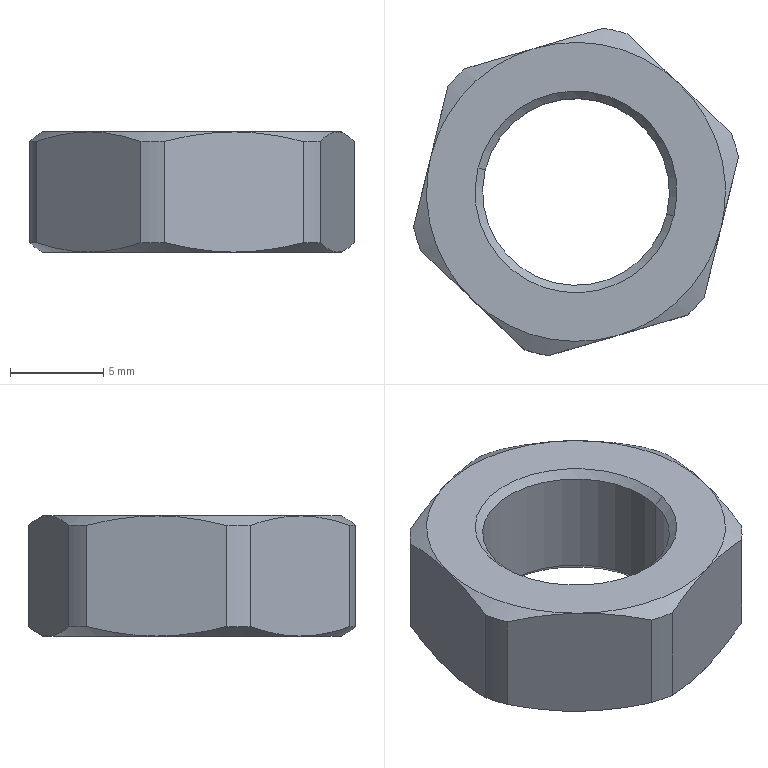Component | SolidWorks | ControlAssembly-1_UWAFN120-1_3_1-1 | 1 solid | 32 faces | box 17.38 x 17.53 x 6.43 mm | volume 899 mm3 | cone 16 | cylinder 8 | plane 8 | commonest cylinder face diameters 17.77 x6 10.002 x2
STEP:
#1=CARTESIAN_POINT('',(24.816,0.7631,20.553));
#2=VERTEX_POINT('',#1);
#3=CARTESIAN_POINT('',(24.433,0.8563,20.553));
#4=VERTEX_POINT('',#3);
#5=CARTESIAN_POINT('',(24.624,0.8097,20.553));
#6=DIRECTION('',(-0.00009864,0.,-1.));
#7=DIRECTION('',(-0.9716,0.2366,0.00009584));
#8=AXIS2_PLACEMENT_3D('',#5,#6,#7);
#9=CIRCLE('',#8,0.1969);
#10=EDGE_CURVE('',#2,#4,#9,.T.);
#11=ORIENTED_EDGE('',*,*,#10,.T.);
#12=CARTESIAN_POINT('',(24.418,0.86,20.569));
#13=VERTEX_POINT('',#12);
#14=CARTESIAN_POINT('',(24.433,0.8563,20.553));
#15=DIRECTION('',(-0.687,0.1673,0.7072));
#16=VECTOR('',#15,39.37);
#17=LINE('',#14,#16);
#18=EDGE_CURVE('',#4,#13,#17,.T.);
#19=ORIENTED_EDGE('',*,*,#18,.T.);
#20=CARTESIAN_POINT('',(24.831,0.7594,20.569));
#21=VERTEX_POINT('',#20);
#22=CARTESIAN_POINT('',(24.624,0.8097,20.569));
#23=DIRECTION('',(0.00009864,-0.,1.));
#24=DIRECTION('',(0.9716,-0.2366,-0.00009584));
#25=AXIS2_PLACEMENT_3D('',#22,#23,#24);
#26=CIRCLE('',#25,0.2126);
#27=EDGE_CURVE('',#13,#21,#26,.T.);
#28=ORIENTED_EDGE('',*,*,#27,.T.);
#29=CARTESIAN_POINT('',(24.816,0.7631,20.553));
#30=DIRECTION('',(0.6871,-0.1673,0.707));
#31=VECTOR('',#30,39.37);
#32=LINE('',#29,#31);
#33=EDGE_CURVE('',#2,#21,#32,.T.);
#34=ORIENTED_EDGE('',*,*,#33,.F.);
#35=EDGE_LOOP('',(#11,#19,#28,#34));
#36=FACE_OUTER_BOUND('',#35,.T.);
#37=CARTESIAN_POINT('',(24.624,0.8097,20.553));
#38=DIRECTION('',(0.00009864,-0.,1.));
#39=DIRECTION('',(0.9716,-0.2366,-0.00009584));
#40=AXIS2_PLACEMENT_3D('',#37,#38,#39);
#41=CONICAL_SURFACE('',#40,0.1969,0.7854);
#42=ADVANCED_FACE('',(#36),#41,.F.);
#43=ORIENTED_EDGE('',*,*,#10,.F.);
#44=CARTESIAN_POINT('',(24.816,0.7631,20.331));
#45=VERTEX_POINT('',#44);
#46=CARTESIAN_POINT('',(24.816,0.7631,20.198));
#47=DIRECTION('',(-0.00009864,0.,-1.));
#48=VECTOR('',#47,39.37);
#49=LINE('',#46,#48);
#50=EDGE_CURVE('',#2,#45,#49,.T.);
#51=ORIENTED_EDGE('',*,*,#50,.T.);
#52=CARTESIAN_POINT('',(24.433,0.8563,20.331));
#53=VERTEX_POINT('',#52);
#54=CARTESIAN_POINT('',(24.624,0.8097,20.331));
#55=DIRECTION('',(-0.00009864,0.,-1.));
#56=DIRECTION('',(-0.9716,0.2366,0.00009584));
#57=AXIS2_PLACEMENT_3D('',#54,#55,#56);
#58=CIRCLE('',#57,0.1969);
#59=EDGE_CURVE('',#45,#53,#58,.T.);
#60=ORIENTED_EDGE('',*,*,#59,.T.);
#61=CARTESIAN_POINT('',(24.433,0.8563,20.198));
#62=DIRECTION('',(-0.00009864,0.,-1.));
#63=VECTOR('',#62,39.37);
#64=LINE('',#61,#63);
#65=EDGE_CURVE('',#4,#53,#64,.T.);
#66=ORIENTED_EDGE('',*,*,#65,.F.);
#67=EDGE_LOOP('',(#43,#51,#60,#66));
#68=FACE_OUTER_BOUND('',#67,.T.);
#69=CARTESIAN_POINT('',(24.624,0.8097,20.198));
#70=DIRECTION('',(-0.00009864,0.,-1.));
#71=DIRECTION('',(-0.9716,0.2366,0.00009584));
#72=AXIS2_PLACEMENT_3D('',#69,#70,#71);
#73=CYLINDRICAL_SURFACE('',#72,0.1969);
#74=ADVANCED_FACE('',(#68),#73,.F.);
#75=ORIENTED_EDGE('',*,*,#59,.F.);
#76=CARTESIAN_POINT('',(24.831,0.7594,20.316));
#77=VERTEX_POINT('',#76);
#78=CARTESIAN_POINT('',(24.869,0.7501,20.276));
#79=DIRECTION('',(0.687,-0.1673,-0.7072));
#80=VECTOR('',#79,39.37);
#81=LINE('',#78,#80);
#82=EDGE_CURVE('',#45,#77,#81,.T.);
#83=ORIENTED_EDGE('',*,*,#82,.T.);
#84=CARTESIAN_POINT('',(24.418,0.86,20.316));
#85=VERTEX_POINT('',#84);
#86=CARTESIAN_POINT('',(24.624,0.8097,20.316));
#87=DIRECTION('',(-0.00009864,0.,-1.));
#88=DIRECTION('',(-0.9716,0.2366,0.00009584));
#89=AXIS2_PLACEMENT_3D('',#86,#87,#88);
#90=CIRCLE('',#89,0.2126);
#91=EDGE_CURVE('',#77,#85,#90,.T.);
#92=ORIENTED_EDGE('',*,*,#91,.T.);
#93=CARTESIAN_POINT('',(24.379,0.8693,20.276));
#94=DIRECTION('',(-0.6871,0.1673,-0.707));
#95=VECTOR('',#94,39.37);
#96=LINE('',#93,#95);
#97=EDGE_CURVE('',#53,#85,#96,.T.);
#98=ORIENTED_EDGE('',*,*,#97,.F.);
#99=EDGE_LOOP('',(#75,#83,#92,#98));
#100=FACE_OUTER_BOUND('',#99,.T.);
#101=CARTESIAN_POINT('',(24.624,0.8097,20.276));
#102=DIRECTION('',(-0.00009864,0.,-1.));
#103=DIRECTION('',(-0.9716,0.2366,0.00009584));
#104=AXIS2_PLACEMENT_3D('',#101,#102,#103);
#105=CONICAL_SURFACE('',#104,0.252,0.7854);
#106=ADVANCED_FACE('',(#100),#105,.F.);
#107=CARTESIAN_POINT('',(24.624,0.8097,20.316));
#108=DIRECTION('',(-0.00009864,0.,-1.));
#109=DIRECTION('',(-0.9716,0.2366,0.00009584));
#110=AXIS2_PLACEMENT_3D('',#107,#108,#109);
#111=CIRCLE('',#110,0.2126);
#112=EDGE_CURVE('',#85,#77,#111,.T.);
#113=ORIENTED_EDGE('',*,*,#112,.F.);
#114=ORIENTED_EDGE('',*,*,#91,.F.);
#115=EDGE_LOOP('',(#113,#114));
#116=FACE_BOUND('',#115,.T.);
#117=CARTESIAN_POINT('',(24.842,1.037,20.316));
#118=VERTEX_POINT('',#117);
#119=CARTESIAN_POINT('',(24.93,0.7352,20.316));
#120=VERTEX_POINT('',#119);
#121=CARTESIAN_POINT('',(24.624,0.8097,20.316));
#122=DIRECTION('',(-0.00009864,0.,-1.));
#123=DIRECTION('',(0.9716,-0.2366,-0.00009584));
#124=AXIS2_PLACEMENT_3D('',#121,#122,#123);
#125=CIRCLE('',#124,0.315);
#126=EDGE_CURVE('',#118,#120,#125,.T.);
#127=ORIENTED_EDGE('',*,*,#126,.T.);
#128=CARTESIAN_POINT('',(24.713,0.5074,20.316));
#129=VERTEX_POINT('',#128);
#130=CARTESIAN_POINT('',(24.624,0.8097,20.316));
#131=DIRECTION('',(-0.00009864,0.,-1.));
#132=DIRECTION('',(0.9716,-0.2366,-0.00009584));
#133=AXIS2_PLACEMENT_3D('',#130,#131,#132);
#134=CIRCLE('',#133,0.315);
#135=EDGE_CURVE('',#120,#129,#134,.T.);
#136=ORIENTED_EDGE('',*,*,#135,.T.);
#137=CARTESIAN_POINT('',(24.407,0.5819,20.316));
#138=VERTEX_POINT('',#137);
#139=CARTESIAN_POINT('',(24.624,0.8097,20.316));
#140=DIRECTION('',(-0.00009864,0.,-1.));
#141=DIRECTION('',(0.9716,-0.2366,-0.00009584));
#142=AXIS2_PLACEMENT_3D('',#139,#140,#141);
#143=CIRCLE('',#142,0.315);
#144=EDGE_CURVE('',#129,#138,#143,.T.);
#145=ORIENTED_EDGE('',*,*,#144,.T.);
#146=CARTESIAN_POINT('',(24.318,0.8842,20.316));
#147=VERTEX_POINT('',#146);
#148=CARTESIAN_POINT('',(24.624,0.8097,20.316));
#149=DIRECTION('',(-0.00009864,0.,-1.));
#150=DIRECTION('',(0.9716,-0.2366,-0.00009584));
#151=AXIS2_PLACEMENT_3D('',#148,#149,#150);
#152=CIRCLE('',#151,0.315);
#153=EDGE_CURVE('',#138,#147,#152,.T.);
#154=ORIENTED_EDGE('',*,*,#153,.T.);
#155=CARTESIAN_POINT('',(24.536,1.112,20.316));
#156=VERTEX_POINT('',#155);
#157=CARTESIAN_POINT('',(24.624,0.8097,20.316));
#158=DIRECTION('',(-0.00009864,0.,-1.));
#159=DIRECTION('',(0.9716,-0.2366,-0.00009584));
#160=AXIS2_PLACEMENT_3D('',#157,#158,#159);
#161=CIRCLE('',#160,0.315);
#162=EDGE_CURVE('',#147,#156,#161,.T.);
#163=ORIENTED_EDGE('',*,*,#162,.T.);
#164=CARTESIAN_POINT('',(24.624,0.8097,20.316));
#165=DIRECTION('',(-0.00009864,0.,-1.));
#166=DIRECTION('',(0.9716,-0.2366,-0.00009584));
#167=AXIS2_PLACEMENT_3D('',#164,#165,#166);
#168=CIRCLE('',#167,0.315);
#169=EDGE_CURVE('',#156,#118,#168,.T.);
#170=ORIENTED_EDGE('',*,*,#169,.T.);
#171=EDGE_LOOP('',(#127,#136,#145,#154,#163,#170));
#172=FACE_OUTER_BOUND('',#171,.T.);
#173=CARTESIAN_POINT('',(24.587,0.6567,20.316));
#174=DIRECTION('',(-0.00009864,0.,-1.));
#175=DIRECTION('',(-0.9716,0.2366,0.00009584));
#176=AXIS2_PLACEMENT_3D('',#173,#174,#175);
#177=PLANE('',#176);
#178=ADVANCED_FACE('',(#116,#172),#177,.T.);
#179=CARTESIAN_POINT('',(24.859,0.5502,20.336));
#180=VERTEX_POINT('',#179);
#181=CARTESIAN_POINT('',(24.859,0.5502,20.336));
#182=CARTESIAN_POINT('',(24.811,0.5361,20.323));
#183=CARTESIAN_POINT('',(24.762,0.5219,20.316));
#184=CARTESIAN_POINT('',(24.713,0.5074,20.316));
#185=B_SPLINE_CURVE_WITH_KNOTS('',3,(#181,#182,#183,#184),.UNSPECIFIED.,.F.,.F.,(4,4),(0.,0.003899),.UNSPECIFIED.);
#186=EDGE_CURVE('',#180,#129,#185,.T.);
#187=ORIENTED_EDGE('',*,*,#186,.T.);
#188=ORIENTED_EDGE('',*,*,#135,.F.);
#189=CARTESIAN_POINT('',(24.894,0.5873,20.336));
#190=VERTEX_POINT('',#189);
#191=CARTESIAN_POINT('',(24.93,0.7352,20.316));
#192=CARTESIAN_POINT('',(24.918,0.685,20.316));
#193=CARTESIAN_POINT('',(24.906,0.6358,20.323));
#194=CARTESIAN_POINT('',(24.894,0.5873,20.336));
#195=B_SPLINE_CURVE_WITH_KNOTS('',3,(#191,#192,#193,#194),.UNSPECIFIED.,.F.,.F.,(4,4),(0.,0.003899),.UNSPECIFIED.);
#196=EDGE_CURVE('',#120,#190,#195,.T.);
#197=ORIENTED_EDGE('',*,*,#196,.T.);
#198=CARTESIAN_POINT('',(24.624,0.8097,20.336));
#199=DIRECTION('',(0.00009864,-0.,1.));
#200=DIRECTION('',(0.9716,-0.2366,-0.00009584));
#201=AXIS2_PLACEMENT_3D('',#198,#199,#200);
#202=CIRCLE('',#201,0.3498);
#203=EDGE_CURVE('',#180,#190,#202,.T.);
#204=ORIENTED_EDGE('',*,*,#203,.F.);
#205=EDGE_LOOP('',(#187,#188,#197,#204));
#206=FACE_OUTER_BOUND('',#205,.T.);
#207=CARTESIAN_POINT('',(24.624,0.8097,20.336));
#208=DIRECTION('',(0.00009864,-0.,1.));
#209=DIRECTION('',(0.9716,-0.2366,-0.00009584));
#210=AXIS2_PLACEMENT_3D('',#207,#208,#209);
#211=CONICAL_SURFACE('',#210,0.3498,1.047);
#212=ADVANCED_FACE('',(#206),#211,.T.);
#213=CARTESIAN_POINT('',(24.952,0.9323,20.336));
#214=VERTEX_POINT('',#213);
#215=CARTESIAN_POINT('',(24.842,1.037,20.316));
#216=CARTESIAN_POINT('',(24.879,1.002,20.316));
#217=CARTESIAN_POINT('',(24.916,0.9668,20.323));
#218=CARTESIAN_POINT('',(24.952,0.9323,20.336));
#219=B_SPLINE_CURVE_WITH_KNOTS('',3,(#215,#216,#217,#218),.UNSPECIFIED.,.F.,.F.,(4,4),(0.,0.003899),.UNSPECIFIED.);
#220=EDGE_CURVE('',#118,#214,#219,.T.);
#221=ORIENTED_EDGE('',*,*,#220,.T.);
#222=CARTESIAN_POINT('',(24.966,0.883,20.336));
#223=VERTEX_POINT('',#222);
#224=CARTESIAN_POINT('',(24.624,0.8097,20.336));
#225=DIRECTION('',(0.00009864,-0.,1.));
#226=DIRECTION('',(0.9716,-0.2366,-0.00009584));
#227=AXIS2_PLACEMENT_3D('',#224,#225,#226);
#228=CIRCLE('',#227,0.3498);
#229=EDGE_CURVE('',#223,#214,#228,.T.);
#230=ORIENTED_EDGE('',*,*,#229,.F.);
#231=CARTESIAN_POINT('',(24.966,0.883,20.336));
#232=CARTESIAN_POINT('',(24.954,0.8345,20.323));
#233=CARTESIAN_POINT('',(24.942,0.7853,20.316));
#234=CARTESIAN_POINT('',(24.93,0.7352,20.316));
#235=B_SPLINE_CURVE_WITH_KNOTS('',3,(#231,#232,#233,#234),.UNSPECIFIED.,.F.,.F.,(4,4),(0.,0.003899),.UNSPECIFIED.);
#236=EDGE_CURVE('',#223,#120,#235,.T.);
#237=ORIENTED_EDGE('',*,*,#236,.T.);
#238=ORIENTED_EDGE('',*,*,#126,.F.);
#239=EDGE_LOOP('',(#221,#230,#237,#238));
#240=FACE_OUTER_BOUND('',#239,.T.);
#241=CARTESIAN_POINT('',(24.624,0.8097,20.336));
#242=DIRECTION('',(0.00009864,-0.,1.));
#243=DIRECTION('',(0.9716,-0.2366,-0.00009584));
#244=AXIS2_PLACEMENT_3D('',#241,#242,#243);
#245=CONICAL_SURFACE('',#244,0.3498,1.047);
#246=ADVANCED_FACE('',(#240),#245,.T.);
#247=CARTESIAN_POINT('',(24.732,1.143,20.336));
#248=VERTEX_POINT('',#247);
#249=CARTESIAN_POINT('',(24.732,1.143,20.336));
#250=CARTESIAN_POINT('',(24.768,1.108,20.323));
#251=CARTESIAN_POINT('',(24.804,1.073,20.316));
#252=CARTESIAN_POINT('',(24.842,1.037,20.316));
#253=B_SPLINE_CURVE_WITH_KNOTS('',3,(#249,#250,#251,#252),.UNSPECIFIED.,.F.,.F.,(4,4),(0.,0.003899),.UNSPECIFIED.);
#254=EDGE_CURVE('',#248,#118,#253,.T.);
#255=ORIENTED_EDGE('',*,*,#254,.T.);
#256=ORIENTED_EDGE('',*,*,#169,.F.);
#257=CARTESIAN_POINT('',(24.682,1.155,20.336));
#258=VERTEX_POINT('',#257);
#259=CARTESIAN_POINT('',(24.536,1.112,20.316));
#260=CARTESIAN_POINT('',(24.585,1.126,20.316));
#261=CARTESIAN_POINT('',(24.634,1.141,20.323));
#262=CARTESIAN_POINT('',(24.682,1.155,20.336));
#263=B_SPLINE_CURVE_WITH_KNOTS('',3,(#259,#260,#261,#262),.UNSPECIFIED.,.F.,.F.,(4,4),(0.,0.003899),.UNSPECIFIED.);
#264=EDGE_CURVE('',#156,#258,#263,.T.);
#265=ORIENTED_EDGE('',*,*,#264,.T.);
#266=CARTESIAN_POINT('',(24.624,0.8097,20.336));
#267=DIRECTION('',(0.00009864,-0.,1.));
#268=DIRECTION('',(0.9716,-0.2366,-0.00009584));
#269=AXIS2_PLACEMENT_3D('',#266,#267,#268);
#270=CIRCLE('',#269,0.3498);
#271=EDGE_CURVE('',#248,#258,#270,.T.);
#272=ORIENTED_EDGE('',*,*,#271,.F.);
#273=EDGE_LOOP('',(#255,#256,#265,#272));
#274=FACE_OUTER_BOUND('',#273,.T.);
#275=CARTESIAN_POINT('',(24.624,0.8097,20.336));
#276=DIRECTION('',(0.00009864,-0.,1.));
#277=DIRECTION('',(0.9716,-0.2366,-0.00009584));
#278=AXIS2_PLACEMENT_3D('',#275,#276,#277);
#279=CONICAL_SURFACE('',#278,0.3498,1.047);
#280=ADVANCED_FACE('',(#274),#279,.T.);
#281=CARTESIAN_POINT('',(24.354,1.032,20.336));
#282=VERTEX_POINT('',#281);
#283=CARTESIAN_POINT('',(24.318,0.8842,20.316));
#284=CARTESIAN_POINT('',(24.33,0.9344,20.316));
#285=CARTESIAN_POINT('',(24.342,0.9836,20.323));
#286=CARTESIAN_POINT('',(24.354,1.032,20.336));
#287=B_SPLINE_CURVE_WITH_KNOTS('',3,(#283,#284,#285,#286),.UNSPECIFIED.,.F.,.F.,(4,4),(0.,0.003899),.UNSPECIFIED.);
#288=EDGE_CURVE('',#147,#282,#287,.T.);
#289=ORIENTED_EDGE('',*,*,#288,.T.);
#290=CARTESIAN_POINT('',(24.39,1.069,20.336));
#291=VERTEX_POINT('',#290);
#292=CARTESIAN_POINT('',(24.624,0.8097,20.336));
#293=DIRECTION('',(0.00009864,-0.,1.));
#294=DIRECTION('',(0.9716,-0.2366,-0.00009584));
#295=AXIS2_PLACEMENT_3D('',#292,#293,#294);
#296=CIRCLE('',#295,0.3498);
#297=EDGE_CURVE('',#291,#282,#296,.T.);
#298=ORIENTED_EDGE('',*,*,#297,.F.);
#299=CARTESIAN_POINT('',(24.39,1.069,20.336));
#300=CARTESIAN_POINT('',(24.438,1.083,20.323));
#301=CARTESIAN_POINT('',(24.486,1.097,20.316));
#302=CARTESIAN_POINT('',(24.536,1.112,20.316));
#303=B_SPLINE_CURVE_WITH_KNOTS('',3,(#299,#300,#301,#302),.UNSPECIFIED.,.F.,.F.,(4,4),(0.,0.003899),.UNSPECIFIED.);
#304=EDGE_CURVE('',#291,#156,#303,.T.);
#305=ORIENTED_EDGE('',*,*,#304,.T.);
#306=ORIENTED_EDGE('',*,*,#162,.F.);
#307=EDGE_LOOP('',(#289,#298,#305,#306));
#308=FACE_OUTER_BOUND('',#307,.T.);
#309=CARTESIAN_POINT('',(24.624,0.8097,20.336));
#310=DIRECTION('',(0.00009864,-0.,1.));
#311=DIRECTION('',(0.9716,-0.2366,-0.00009584));
#312=AXIS2_PLACEMENT_3D('',#309,#310,#311);
#313=CONICAL_SURFACE('',#312,0.3498,1.047);
#314=ADVANCED_FACE('',(#308),#313,.T.);
#315=CARTESIAN_POINT('',(24.297,0.6871,20.336));
#316=VERTEX_POINT('',#315);
#317=CARTESIAN_POINT('',(24.407,0.5819,20.316));
#318=CARTESIAN_POINT('',(24.369,0.6176,20.316));
#319=CARTESIAN_POINT('',(24.333,0.6526,20.323));
#320=CARTESIAN_POINT('',(24.297,0.6871,20.336));
#321=B_SPLINE_CURVE_WITH_KNOTS('',3,(#317,#318,#319,#320),.UNSPECIFIED.,.F.,.F.,(4,4),(0.,0.003899),.UNSPECIFIED.);
#322=EDGE_CURVE('',#138,#316,#321,.T.);
#323=ORIENTED_EDGE('',*,*,#322,.T.);
#324=CARTESIAN_POINT('',(24.282,0.7364,20.336));
#325=VERTEX_POINT('',#324);
#326=CARTESIAN_POINT('',(24.624,0.8097,20.336));
#327=DIRECTION('',(0.00009864,-0.,1.));
#328=DIRECTION('',(0.9716,-0.2366,-0.00009584));
#329=AXIS2_PLACEMENT_3D('',#326,#327,#328);
#330=CIRCLE('',#329,0.3498);
#331=EDGE_CURVE('',#325,#316,#330,.T.);
#332=ORIENTED_EDGE('',*,*,#331,.F.);
#333=CARTESIAN_POINT('',(24.282,0.7364,20.336));
#334=CARTESIAN_POINT('',(24.294,0.7849,20.323));
#335=CARTESIAN_POINT('',(24.306,0.8341,20.316));
#336=CARTESIAN_POINT('',(24.318,0.8842,20.316));
#337=B_SPLINE_CURVE_WITH_KNOTS('',3,(#333,#334,#335,#336),.UNSPECIFIED.,.F.,.F.,(4,4),(0.,0.003899),.UNSPECIFIED.);
#338=EDGE_CURVE('',#325,#147,#337,.T.);
#339=ORIENTED_EDGE('',*,*,#338,.T.);
#340=ORIENTED_EDGE('',*,*,#153,.F.);
#341=EDGE_LOOP('',(#323,#332,#339,#340));
#342=FACE_OUTER_BOUND('',#341,.T.);
#343=CARTESIAN_POINT('',(24.624,0.8097,20.336));
#344=DIRECTION('',(0.00009864,-0.,1.));
#345=DIRECTION('',(0.9716,-0.2366,-0.00009584));
#346=AXIS2_PLACEMENT_3D('',#343,#344,#345);
#347=CONICAL_SURFACE('',#346,0.3498,1.047);
#348=ADVANCED_FACE('',(#342),#347,.T.);
#349=CARTESIAN_POINT('',(24.517,0.4768,20.336));
#350=VERTEX_POINT('',#349);
#351=CARTESIAN_POINT('',(24.517,0.4768,20.336));
#352=CARTESIAN_POINT('',(24.481,0.5113,20.323));
#353=CARTESIAN_POINT('',(24.444,0.5463,20.316));
#354=CARTESIAN_POINT('',(24.407,0.5819,20.316));
#355=B_SPLINE_CURVE_WITH_KNOTS('',3,(#351,#352,#353,#354),.UNSPECIFIED.,.F.,.F.,(4,4),(0.,0.003899),.UNSPECIFIED.);
#356=EDGE_CURVE('',#350,#138,#355,.T.);
#357=ORIENTED_EDGE('',*,*,#356,.T.);
#358=ORIENTED_EDGE('',*,*,#144,.F.);
#359=CARTESIAN_POINT('',(24.567,0.4647,20.336));
#360=VERTEX_POINT('',#359);
#361=CARTESIAN_POINT('',(24.713,0.5074,20.316));
#362=CARTESIAN_POINT('',(24.663,0.4929,20.316));
#363=CARTESIAN_POINT('',(24.615,0.4787,20.323));
#364=CARTESIAN_POINT('',(24.567,0.4647,20.336));
#365=B_SPLINE_CURVE_WITH_KNOTS('',3,(#361,#362,#363,#364),.UNSPECIFIED.,.F.,.F.,(4,4),(0.,0.003899),.UNSPECIFIED.);
#366=EDGE_CURVE('',#129,#360,#365,.T.);
#367=ORIENTED_EDGE('',*,*,#366,.T.);
#368=CARTESIAN_POINT('',(24.624,0.8097,20.336));
#369=DIRECTION('',(0.00009864,-0.,1.));
#370=DIRECTION('',(0.9716,-0.2366,-0.00009584));
#371=AXIS2_PLACEMENT_3D('',#368,#369,#370);
#372=CIRCLE('',#371,0.3498);
#373=EDGE_CURVE('',#350,#360,#372,.T.);
#374=ORIENTED_EDGE('',*,*,#373,.F.);
#375=EDGE_LOOP('',(#357,#358,#367,#374));
#376=FACE_OUTER_BOUND('',#375,.T.);
#377=CARTESIAN_POINT('',(24.624,0.8097,20.336));
#378=DIRECTION('',(0.00009864,-0.,1.));
#379=DIRECTION('',(0.9716,-0.2366,-0.00009584));
#380=AXIS2_PLACEMENT_3D('',#377,#378,#379);
#381=CONICAL_SURFACE('',#380,0.3498,1.047);
#382=ADVANCED_FACE('',(#376),#381,.T.);
#383=CARTESIAN_POINT('',(24.567,0.4647,20.549));
#384=VERTEX_POINT('',#383);
#385=CARTESIAN_POINT('',(24.713,0.5074,20.569));
#386=VERTEX_POINT('',#385);
#387=CARTESIAN_POINT('',(24.567,0.4647,20.549));
#388=CARTESIAN_POINT('',(24.615,0.4787,20.561));
#389=CARTESIAN_POINT('',(24.663,0.4929,20.569));
#390=CARTESIAN_POINT('',(24.713,0.5074,20.569));
#391=B_SPLINE_CURVE_WITH_KNOTS('',3,(#387,#388,#389,#390),.UNSPECIFIED.,.F.,.F.,(4,4),(0.,0.003899),.UNSPECIFIED.);
#392=EDGE_CURVE('',#384,#386,#391,.T.);
#393=ORIENTED_EDGE('',*,*,#392,.F.);
#394=CARTESIAN_POINT('',(24.567,0.4647,20.316));
#395=DIRECTION('',(0.00009864,-0.,1.));
#396=VECTOR('',#395,39.37);
#397=LINE('',#394,#396);
#398=EDGE_CURVE('',#360,#384,#397,.T.);
#399=ORIENTED_EDGE('',*,*,#398,.F.);
#400=ORIENTED_EDGE('',*,*,#366,.F.);
#401=ORIENTED_EDGE('',*,*,#186,.F.);
#402=CARTESIAN_POINT('',(24.859,0.5502,20.549));
#403=VERTEX_POINT('',#402);
#404=CARTESIAN_POINT('',(24.859,0.5502,20.316));
#405=DIRECTION('',(-0.00009864,0.,-1.));
#406=VECTOR('',#405,39.37);
#407=LINE('',#404,#406);
#408=EDGE_CURVE('',#403,#180,#407,.T.);
#409=ORIENTED_EDGE('',*,*,#408,.F.);
#410=CARTESIAN_POINT('',(24.713,0.5074,20.569));
#411=CARTESIAN_POINT('',(24.762,0.5219,20.569));
#412=CARTESIAN_POINT('',(24.811,0.5361,20.561));
#413=CARTESIAN_POINT('',(24.859,0.5502,20.549));
#414=B_SPLINE_CURVE_WITH_KNOTS('',3,(#410,#411,#412,#413),.UNSPECIFIED.,.F.,.F.,(4,4),(0.,0.003899),.UNSPECIFIED.);
#415=EDGE_CURVE('',#386,#403,#414,.T.);
#416=ORIENTED_EDGE('',*,*,#415,.F.);
#417=EDGE_LOOP('',(#393,#399,#400,#401,#409,#416));
#418=FACE_OUTER_BOUND('',#417,.T.);
#419=CARTESIAN_POINT('',(24.538,0.4563,20.316));
#420=DIRECTION('',(-0.2809,0.9597,0.00002771));
#421=DIRECTION('',(-0.9597,-0.2809,0.00009467));
#422=AXIS2_PLACEMENT_3D('',#419,#420,#421);
#423=PLANE('',#422);
#424=ADVANCED_FACE('',(#418),#423,.F.);
#425=CARTESIAN_POINT('',(24.894,0.5873,20.549));
#426=VERTEX_POINT('',#425);
#427=CARTESIAN_POINT('',(24.93,0.7352,20.569));
#428=VERTEX_POINT('',#427);
#429=CARTESIAN_POINT('',(24.894,0.5873,20.549));
#430=CARTESIAN_POINT('',(24.906,0.6358,20.561));
#431=CARTESIAN_POINT('',(24.918,0.685,20.569));
#432=CARTESIAN_POINT('',(24.93,0.7352,20.569));
#433=B_SPLINE_CURVE_WITH_KNOTS('',3,(#429,#430,#431,#432),.UNSPECIFIED.,.F.,.F.,(4,4),(0.,0.003899),.UNSPECIFIED.);
#434=EDGE_CURVE('',#426,#428,#433,.T.);
#435=ORIENTED_EDGE('',*,*,#434,.F.);
#436=CARTESIAN_POINT('',(24.894,0.5873,20.316));
#437=DIRECTION('',(0.00009864,-0.,1.));
#438=VECTOR('',#437,39.37);
#439=LINE('',#436,#438);
#440=EDGE_CURVE('',#190,#426,#439,.T.);
#441=ORIENTED_EDGE('',*,*,#440,.F.);
#442=ORIENTED_EDGE('',*,*,#196,.F.);
#443=ORIENTED_EDGE('',*,*,#236,.F.);
#444=CARTESIAN_POINT('',(24.966,0.883,20.549));
#445=VERTEX_POINT('',#444);
#446=CARTESIAN_POINT('',(24.966,0.883,20.316));
#447=DIRECTION('',(-0.00009864,0.,-1.));
#448=VECTOR('',#447,39.37);
#449=LINE('',#446,#448);
#450=EDGE_CURVE('',#445,#223,#449,.T.);
#451=ORIENTED_EDGE('',*,*,#450,.F.);
#452=CARTESIAN_POINT('',(24.93,0.7352,20.569));
#453=CARTESIAN_POINT('',(24.942,0.7853,20.569));
#454=CARTESIAN_POINT('',(24.954,0.8345,20.561));
#455=CARTESIAN_POINT('',(24.966,0.883,20.549));
#456=B_SPLINE_CURVE_WITH_KNOTS('',3,(#452,#453,#454,#455),.UNSPECIFIED.,.F.,.F.,(4,4),(0.,0.003899),.UNSPECIFIED.);
#457=EDGE_CURVE('',#428,#445,#456,.T.);
#458=ORIENTED_EDGE('',*,*,#457,.F.);
#459=EDGE_LOOP('',(#435,#441,#442,#443,#451,#458));
#460=FACE_OUTER_BOUND('',#459,.T.);
#461=CARTESIAN_POINT('',(24.887,0.5585,20.316));
#462=DIRECTION('',(-0.9716,0.2366,0.00009584));
#463=DIRECTION('',(-0.2366,-0.9716,0.00002334));
#464=AXIS2_PLACEMENT_3D('',#461,#462,#463);
#465=PLANE('',#464);
#466=ADVANCED_FACE('',(#460),#465,.F.);
#467=CARTESIAN_POINT('',(24.952,0.9323,20.549));
#468=VERTEX_POINT('',#467);
#469=CARTESIAN_POINT('',(24.842,1.037,20.569));
#470=VERTEX_POINT('',#469);
#471=CARTESIAN_POINT('',(24.952,0.9323,20.549));
#472=CARTESIAN_POINT('',(24.916,0.9668,20.561));
#473=CARTESIAN_POINT('',(24.879,1.002,20.569));
#474=CARTESIAN_POINT('',(24.842,1.037,20.569));
#475=B_SPLINE_CURVE_WITH_KNOTS('',3,(#471,#472,#473,#474),.UNSPECIFIED.,.F.,.F.,(4,4),(0.,0.003899),.UNSPECIFIED.);
#476=EDGE_CURVE('',#468,#470,#475,.T.);
#477=ORIENTED_EDGE('',*,*,#476,.F.);
#478=CARTESIAN_POINT('',(24.952,0.9323,20.316));
#479=DIRECTION('',(0.00009864,-0.,1.));
#480=VECTOR('',#479,39.37);
#481=LINE('',#478,#480);
#482=EDGE_CURVE('',#214,#468,#481,.T.);
#483=ORIENTED_EDGE('',*,*,#482,.F.);
#484=ORIENTED_EDGE('',*,*,#220,.F.);
#485=ORIENTED_EDGE('',*,*,#254,.F.);
#486=CARTESIAN_POINT('',(24.732,1.143,20.549));
#487=VERTEX_POINT('',#486);
#488=CARTESIAN_POINT('',(24.732,1.143,20.316));
#489=DIRECTION('',(-0.00009864,0.,-1.));
#490=VECTOR('',#489,39.37);
#491=LINE('',#488,#490);
#492=EDGE_CURVE('',#487,#248,#491,.T.);
#493=ORIENTED_EDGE('',*,*,#492,.F.);
#494=CARTESIAN_POINT('',(24.842,1.037,20.569));
#495=CARTESIAN_POINT('',(24.804,1.073,20.569));
#496=CARTESIAN_POINT('',(24.768,1.108,20.561));
#497=CARTESIAN_POINT('',(24.732,1.143,20.549));
#498=B_SPLINE_CURVE_WITH_KNOTS('',3,(#494,#495,#496,#497),.UNSPECIFIED.,.F.,.F.,(4,4),(0.,0.003899),.UNSPECIFIED.);
#499=EDGE_CURVE('',#470,#487,#498,.T.);
#500=ORIENTED_EDGE('',*,*,#499,.F.);
#501=EDGE_LOOP('',(#477,#483,#484,#485,#493,#500));
#502=FACE_OUTER_BOUND('',#501,.T.);
#503=CARTESIAN_POINT('',(24.973,0.9119,20.316));
#504=DIRECTION('',(-0.6907,-0.7231,0.00006814));
#505=DIRECTION('',(0.7231,-0.6907,-0.00007133));
#506=AXIS2_PLACEMENT_3D('',#503,#504,#505);
#507=PLANE('',#506);
#508=ADVANCED_FACE('',(#502),#507,.F.);
#509=CARTESIAN_POINT('',(24.682,1.155,20.549));
#510=VERTEX_POINT('',#509);
#511=CARTESIAN_POINT('',(24.536,1.112,20.569));
#512=VERTEX_POINT('',#511);
#513=CARTESIAN_POINT('',(24.682,1.155,20.549));
#514=CARTESIAN_POINT('',(24.634,1.141,20.561));
#515=CARTESIAN_POINT('',(24.585,1.126,20.569));
#516=CARTESIAN_POINT('',(24.536,1.112,20.569));
#517=B_SPLINE_CURVE_WITH_KNOTS('',3,(#513,#514,#515,#516),.UNSPECIFIED.,.F.,.F.,(4,4),(0.,0.003899),.UNSPECIFIED.);
#518=EDGE_CURVE('',#510,#512,#517,.T.);
#519=ORIENTED_EDGE('',*,*,#518,.F.);
#520=CARTESIAN_POINT('',(24.682,1.155,20.316));
#521=DIRECTION('',(0.00009864,-0.,1.));
#522=VECTOR('',#521,39.37);
#523=LINE('',#520,#522);
#524=EDGE_CURVE('',#258,#510,#523,.T.);
#525=ORIENTED_EDGE('',*,*,#524,.F.);
#526=ORIENTED_EDGE('',*,*,#264,.F.);
#527=ORIENTED_EDGE('',*,*,#304,.F.);
#528=CARTESIAN_POINT('',(24.39,1.069,20.549));
#529=VERTEX_POINT('',#528);
#530=CARTESIAN_POINT('',(24.39,1.069,20.316));
#531=DIRECTION('',(-0.00009864,0.,-1.));
#532=VECTOR('',#531,39.37);
#533=LINE('',#530,#532);
#534=EDGE_CURVE('',#529,#291,#533,.T.);
#535=ORIENTED_EDGE('',*,*,#534,.F.);
#536=CARTESIAN_POINT('',(24.536,1.112,20.569));
#537=CARTESIAN_POINT('',(24.486,1.097,20.569));
#538=CARTESIAN_POINT('',(24.438,1.083,20.561));
#539=CARTESIAN_POINT('',(24.39,1.069,20.549));
#540=B_SPLINE_CURVE_WITH_KNOTS('',3,(#536,#537,#538,#539),.UNSPECIFIED.,.F.,.F.,(4,4),(0.,0.003899),.UNSPECIFIED.);
#541=EDGE_CURVE('',#512,#529,#540,.T.);
#542=ORIENTED_EDGE('',*,*,#541,.F.);
#543=EDGE_LOOP('',(#519,#525,#526,#527,#535,#542));
#544=FACE_OUTER_BOUND('',#543,.T.);
#545=CARTESIAN_POINT('',(24.71,1.163,20.316));
#546=DIRECTION('',(0.2809,-0.9597,-0.00002771));
#547=DIRECTION('',(0.9597,0.2809,-0.00009467));
#548=AXIS2_PLACEMENT_3D('',#545,#546,#547);
#549=PLANE('',#548);
#550=ADVANCED_FACE('',(#544),#549,.F.);
#551=CARTESIAN_POINT('',(24.354,1.032,20.549));
#552=VERTEX_POINT('',#551);
#553=CARTESIAN_POINT('',(24.318,0.8842,20.569));
#554=VERTEX_POINT('',#553);
#555=CARTESIAN_POINT('',(24.354,1.032,20.549));
#556=CARTESIAN_POINT('',(24.342,0.9836,20.561));
#557=CARTESIAN_POINT('',(24.33,0.9344,20.569));
#558=CARTESIAN_POINT('',(24.318,0.8842,20.569));
#559=B_SPLINE_CURVE_WITH_KNOTS('',3,(#555,#556,#557,#558),.UNSPECIFIED.,.F.,.F.,(4,4),(0.,0.003899),.UNSPECIFIED.);
#560=EDGE_CURVE('',#552,#554,#559,.T.);
#561=ORIENTED_EDGE('',*,*,#560,.F.);
#562=CARTESIAN_POINT('',(24.354,1.032,20.316));
#563=DIRECTION('',(0.00009864,-0.,1.));
#564=VECTOR('',#563,39.37);
#565=LINE('',#562,#564);
#566=EDGE_CURVE('',#282,#552,#565,.T.);
#567=ORIENTED_EDGE('',*,*,#566,.F.);
#568=ORIENTED_EDGE('',*,*,#288,.F.);
#569=ORIENTED_EDGE('',*,*,#338,.F.);
#570=CARTESIAN_POINT('',(24.282,0.7364,20.549));
#571=VERTEX_POINT('',#570);
#572=CARTESIAN_POINT('',(24.282,0.7364,20.316));
#573=DIRECTION('',(-0.00009864,0.,-1.));
#574=VECTOR('',#573,39.37);
#575=LINE('',#572,#574);
#576=EDGE_CURVE('',#571,#325,#575,.T.);
#577=ORIENTED_EDGE('',*,*,#576,.F.);
#578=CARTESIAN_POINT('',(24.318,0.8842,20.569));
#579=CARTESIAN_POINT('',(24.306,0.8341,20.569));
#580=CARTESIAN_POINT('',(24.294,0.7849,20.561));
#581=CARTESIAN_POINT('',(24.282,0.7364,20.549));
#582=B_SPLINE_CURVE_WITH_KNOTS('',3,(#578,#579,#580,#581),.UNSPECIFIED.,.F.,.F.,(4,4),(0.,0.003899),.UNSPECIFIED.);
#583=EDGE_CURVE('',#554,#571,#582,.T.);
#584=ORIENTED_EDGE('',*,*,#583,.F.);
#585=EDGE_LOOP('',(#561,#567,#568,#569,#577,#584));
#586=FACE_OUTER_BOUND('',#585,.T.);
#587=CARTESIAN_POINT('',(24.361,1.061,20.316));
#588=DIRECTION('',(0.9716,-0.2366,-0.00009584));
#589=DIRECTION('',(0.2366,0.9716,-0.00002334));
#590=AXIS2_PLACEMENT_3D('',#587,#588,#589);
#591=PLANE('',#590);
#592=ADVANCED_FACE('',(#586),#591,.F.);
#593=CARTESIAN_POINT('',(24.297,0.6871,20.549));
#594=VERTEX_POINT('',#593);
#595=CARTESIAN_POINT('',(24.407,0.5819,20.569));
#596=VERTEX_POINT('',#595);
#597=CARTESIAN_POINT('',(24.297,0.6871,20.549));
#598=CARTESIAN_POINT('',(24.333,0.6526,20.561));
#599=CARTESIAN_POINT('',(24.369,0.6176,20.569));
#600=CARTESIAN_POINT('',(24.407,0.5819,20.569));
#601=B_SPLINE_CURVE_WITH_KNOTS('',3,(#597,#598,#599,#600),.UNSPECIFIED.,.F.,.F.,(4,4),(0.,0.003899),.UNSPECIFIED.);
#602=EDGE_CURVE('',#594,#596,#601,.T.);
#603=ORIENTED_EDGE('',*,*,#602,.F.);
#604=CARTESIAN_POINT('',(24.297,0.6871,20.316));
#605=DIRECTION('',(0.00009864,-0.,1.));
#606=VECTOR('',#605,39.37);
#607=LINE('',#604,#606);
#608=EDGE_CURVE('',#316,#594,#607,.T.);
#609=ORIENTED_EDGE('',*,*,#608,.F.);
#610=ORIENTED_EDGE('',*,*,#322,.F.);
#611=ORIENTED_EDGE('',*,*,#356,.F.);
#612=CARTESIAN_POINT('',(24.517,0.4768,20.549));
#613=VERTEX_POINT('',#612);
#614=CARTESIAN_POINT('',(24.517,0.4768,20.316));
#615=DIRECTION('',(-0.00009864,0.,-1.));
#616=VECTOR('',#615,39.37);
#617=LINE('',#614,#616);
#618=EDGE_CURVE('',#613,#350,#617,.T.);
#619=ORIENTED_EDGE('',*,*,#618,.F.);
#620=CARTESIAN_POINT('',(24.407,0.5819,20.569));
#621=CARTESIAN_POINT('',(24.444,0.5463,20.569));
#622=CARTESIAN_POINT('',(24.481,0.5113,20.561));
#623=CARTESIAN_POINT('',(24.517,0.4768,20.549));
#624=B_SPLINE_CURVE_WITH_KNOTS('',3,(#620,#621,#622,#623),.UNSPECIFIED.,.F.,.F.,(4,4),(0.,0.003899),.UNSPECIFIED.);
#625=EDGE_CURVE('',#596,#613,#624,.T.);
#626=ORIENTED_EDGE('',*,*,#625,.F.);
#627=EDGE_LOOP('',(#603,#609,#610,#611,#619,#626));
#628=FACE_OUTER_BOUND('',#627,.T.);
#629=CARTESIAN_POINT('',(24.275,0.7075,20.316));
#630=DIRECTION('',(0.6907,0.7231,-0.00006814));
#631=DIRECTION('',(-0.7231,0.6907,0.00007133));
#632=AXIS2_PLACEMENT_3D('',#629,#630,#631);
#633=PLANE('',#632);
#634=ADVANCED_FACE('',(#628),#633,.F.);
#635=ORIENTED_EDGE('',*,*,#415,.T.);
#636=CARTESIAN_POINT('',(24.624,0.8097,20.549));
#637=DIRECTION('',(0.00009864,-0.,1.));
#638=DIRECTION('',(-0.2366,-0.9716,0.00002334));
#639=AXIS2_PLACEMENT_3D('',#636,#637,#638);
#640=CIRCLE('',#639,0.3498);
#641=EDGE_CURVE('',#403,#426,#640,.T.);
#642=ORIENTED_EDGE('',*,*,#641,.T.);
#643=ORIENTED_EDGE('',*,*,#434,.T.);
#644=CARTESIAN_POINT('',(24.624,0.8097,20.569));
#645=DIRECTION('',(-0.00009864,0.,-1.));
#646=DIRECTION('',(-0.9716,0.2366,0.00009584));
#647=AXIS2_PLACEMENT_3D('',#644,#645,#646);
#648=CIRCLE('',#647,0.315);
#649=EDGE_CURVE('',#428,#386,#648,.T.);
#650=ORIENTED_EDGE('',*,*,#649,.T.);
#651=EDGE_LOOP('',(#635,#642,#643,#650));
#652=FACE_OUTER_BOUND('',#651,.T.);
#653=CARTESIAN_POINT('',(24.624,0.8097,20.549));
#654=DIRECTION('',(-0.00009864,0.,-1.));
#655=DIRECTION('',(-0.9716,0.2366,0.00009584));
#656=AXIS2_PLACEMENT_3D('',#653,#654,#655);
#657=CONICAL_SURFACE('',#656,0.3498,1.047);
#658=ADVANCED_FACE('',(#652),#657,.T.);
#659=ORIENTED_EDGE('',*,*,#392,.T.);
#660=CARTESIAN_POINT('',(24.624,0.8097,20.569));
#661=DIRECTION('',(-0.00009864,0.,-1.));
#662=DIRECTION('',(-0.9716,0.2366,0.00009584));
#663=AXIS2_PLACEMENT_3D('',#660,#661,#662);
#664=CIRCLE('',#663,0.315);
#665=EDGE_CURVE('',#386,#596,#664,.T.);
#666=ORIENTED_EDGE('',*,*,#665,.T.);
#667=ORIENTED_EDGE('',*,*,#625,.T.);
#668=CARTESIAN_POINT('',(24.624,0.8097,20.549));
#669=DIRECTION('',(0.00009864,-0.,1.));
#670=DIRECTION('',(-0.2366,-0.9716,0.00002334));
#671=AXIS2_PLACEMENT_3D('',#668,#669,#670);
#672=CIRCLE('',#671,0.3498);
#673=EDGE_CURVE('',#613,#384,#672,.T.);
#674=ORIENTED_EDGE('',*,*,#673,.T.);
#675=EDGE_LOOP('',(#659,#666,#667,#674));
#676=FACE_OUTER_BOUND('',#675,.T.);
#677=CARTESIAN_POINT('',(24.624,0.8097,20.549));
#678=DIRECTION('',(-0.00009864,0.,-1.));
#679=DIRECTION('',(-0.9716,0.2366,0.00009584));
#680=AXIS2_PLACEMENT_3D('',#677,#678,#679);
#681=CONICAL_SURFACE('',#680,0.3498,1.047);
#682=ADVANCED_FACE('',(#676),#681,.T.);
#683=ORIENTED_EDGE('',*,*,#398,.T.);
#684=ORIENTED_EDGE('',*,*,#673,.F.);
#685=ORIENTED_EDGE('',*,*,#618,.T.);
#686=ORIENTED_EDGE('',*,*,#373,.T.);
#687=EDGE_LOOP('',(#683,#684,#685,#686));
#688=FACE_OUTER_BOUND('',#687,.T.);
#689=CARTESIAN_POINT('',(24.624,0.8097,20.442));
#690=DIRECTION('',(0.00009864,-0.,1.));
#691=DIRECTION('',(0.9716,-0.2366,-0.00009584));
#692=AXIS2_PLACEMENT_3D('',#689,#690,#691);
#693=CYLINDRICAL_SURFACE('',#692,0.3498);
#694=ADVANCED_FACE('',(#688),#693,.T.);
#695=ORIENTED_EDGE('',*,*,#408,.T.);
#696=ORIENTED_EDGE('',*,*,#203,.T.);
#697=ORIENTED_EDGE('',*,*,#440,.T.);
#698=ORIENTED_EDGE('',*,*,#641,.F.);
#699=EDGE_LOOP('',(#695,#696,#697,#698));
#700=FACE_OUTER_BOUND('',#699,.T.);
#701=CARTESIAN_POINT('',(24.624,0.8097,20.442));
#702=DIRECTION('',(0.00009864,-0.,1.));
#703=DIRECTION('',(0.9716,-0.2366,-0.00009584));
#704=AXIS2_PLACEMENT_3D('',#701,#702,#703);
#705=CYLINDRICAL_SURFACE('',#704,0.3498);
#706=ADVANCED_FACE('',(#700),#705,.T.);
#707=ORIENTED_EDGE('',*,*,#476,.T.);
#708=CARTESIAN_POINT('',(24.624,0.8097,20.569));
#709=DIRECTION('',(-0.00009864,0.,-1.));
#710=DIRECTION('',(-0.9716,0.2366,0.00009584));
#711=AXIS2_PLACEMENT_3D('',#708,#709,#710);
#712=CIRCLE('',#711,0.315);
#713=EDGE_CURVE('',#470,#428,#712,.T.);
#714=ORIENTED_EDGE('',*,*,#713,.T.);
#715=ORIENTED_EDGE('',*,*,#457,.T.);
#716=CARTESIAN_POINT('',(24.624,0.8097,20.549));
#717=DIRECTION('',(0.00009864,-0.,1.));
#718=DIRECTION('',(-0.2366,-0.9716,0.00002334));
#719=AXIS2_PLACEMENT_3D('',#716,#717,#718);
#720=CIRCLE('',#719,0.3498);
#721=EDGE_CURVE('',#445,#468,#720,.T.);
#722=ORIENTED_EDGE('',*,*,#721,.T.);
#723=EDGE_LOOP('',(#707,#714,#715,#722));
#724=FACE_OUTER_BOUND('',#723,.T.);
#725=CARTESIAN_POINT('',(24.624,0.8097,20.549));
#726=DIRECTION('',(-0.00009864,0.,-1.));
#727=DIRECTION('',(-0.9716,0.2366,0.00009584));
#728=AXIS2_PLACEMENT_3D('',#725,#726,#727);
#729=CONICAL_SURFACE('',#728,0.3498,1.047);
#730=ADVANCED_FACE('',(#724),#729,.T.);
#731=ORIENTED_EDGE('',*,*,#482,.T.);
#732=ORIENTED_EDGE('',*,*,#721,.F.);
#733=ORIENTED_EDGE('',*,*,#450,.T.);
#734=ORIENTED_EDGE('',*,*,#229,.T.);
#735=EDGE_LOOP('',(#731,#732,#733,#734));
#736=FACE_OUTER_BOUND('',#735,.T.);
#737=CARTESIAN_POINT('',(24.624,0.8097,20.442));
#738=DIRECTION('',(0.00009864,-0.,1.));
#739=DIRECTION('',(0.9716,-0.2366,-0.00009584));
#740=AXIS2_PLACEMENT_3D('',#737,#738,#739);
#741=CYLINDRICAL_SURFACE('',#740,0.3498);
#742=ADVANCED_FACE('',(#736),#741,.T.);
#743=ORIENTED_EDGE('',*,*,#499,.T.);
#744=CARTESIAN_POINT('',(24.624,0.8097,20.549));
#745=DIRECTION('',(0.00009864,-0.,1.));
#746=DIRECTION('',(-0.2366,-0.9716,0.00002334));
#747=AXIS2_PLACEMENT_3D('',#744,#745,#746);
#748=CIRCLE('',#747,0.3498);
#749=EDGE_CURVE('',#487,#510,#748,.T.);
#750=ORIENTED_EDGE('',*,*,#749,.T.);
#751=ORIENTED_EDGE('',*,*,#518,.T.);
#752=CARTESIAN_POINT('',(24.624,0.8097,20.569));
#753=DIRECTION('',(-0.00009864,0.,-1.));
#754=DIRECTION('',(-0.9716,0.2366,0.00009584));
#755=AXIS2_PLACEMENT_3D('',#752,#753,#754);
#756=CIRCLE('',#755,0.315);
#757=EDGE_CURVE('',#512,#470,#756,.T.);
#758=ORIENTED_EDGE('',*,*,#757,.T.);
#759=EDGE_LOOP('',(#743,#750,#751,#758));
#760=FACE_OUTER_BOUND('',#759,.T.);
#761=CARTESIAN_POINT('',(24.624,0.8097,20.549));
#762=DIRECTION('',(-0.00009864,0.,-1.));
#763=DIRECTION('',(-0.9716,0.2366,0.00009584));
#764=AXIS2_PLACEMENT_3D('',#761,#762,#763);
#765=CONICAL_SURFACE('',#764,0.3498,1.047);
#766=ADVANCED_FACE('',(#760),#765,.T.);
#767=ORIENTED_EDGE('',*,*,#492,.T.);
#768=ORIENTED_EDGE('',*,*,#271,.T.);
#769=ORIENTED_EDGE('',*,*,#524,.T.);
#770=ORIENTED_EDGE('',*,*,#749,.F.);
#771=EDGE_LOOP('',(#767,#768,#769,#770));
#772=FACE_OUTER_BOUND('',#771,.T.);
#773=CARTESIAN_POINT('',(24.624,0.8097,20.442));
#774=DIRECTION('',(0.00009864,-0.,1.));
#775=DIRECTION('',(0.9716,-0.2366,-0.00009584));
#776=AXIS2_PLACEMENT_3D('',#773,#774,#775);
#777=CYLINDRICAL_SURFACE('',#776,0.3498);
#778=ADVANCED_FACE('',(#772),#777,.T.);
#779=ORIENTED_EDGE('',*,*,#560,.T.);
#780=CARTESIAN_POINT('',(24.624,0.8097,20.569));
#781=DIRECTION('',(-0.00009864,0.,-1.));
#782=DIRECTION('',(-0.9716,0.2366,0.00009584));
#783=AXIS2_PLACEMENT_3D('',#780,#781,#782);
#784=CIRCLE('',#783,0.315);
#785=EDGE_CURVE('',#554,#512,#784,.T.);
#786=ORIENTED_EDGE('',*,*,#785,.T.);
#787=ORIENTED_EDGE('',*,*,#541,.T.);
#788=CARTESIAN_POINT('',(24.624,0.8097,20.549));
#789=DIRECTION('',(0.00009864,-0.,1.));
#790=DIRECTION('',(-0.2366,-0.9716,0.00002334));
#791=AXIS2_PLACEMENT_3D('',#788,#789,#790);
#792=CIRCLE('',#791,0.3498);
#793=EDGE_CURVE('',#529,#552,#792,.T.);
#794=ORIENTED_EDGE('',*,*,#793,.T.);
#795=EDGE_LOOP('',(#779,#786,#787,#794));
#796=FACE_OUTER_BOUND('',#795,.T.);
#797=CARTESIAN_POINT('',(24.624,0.8097,20.549));
#798=DIRECTION('',(-0.00009864,0.,-1.));
#799=DIRECTION('',(-0.9716,0.2366,0.00009584));
#800=AXIS2_PLACEMENT_3D('',#797,#798,#799);
#801=CONICAL_SURFACE('',#800,0.3498,1.047);
#802=ADVANCED_FACE('',(#796),#801,.T.);
#803=ORIENTED_EDGE('',*,*,#566,.T.);
#804=ORIENTED_EDGE('',*,*,#793,.F.);
#805=ORIENTED_EDGE('',*,*,#534,.T.);
#806=ORIENTED_EDGE('',*,*,#297,.T.);
#807=EDGE_LOOP('',(#803,#804,#805,#806));
#808=FACE_OUTER_BOUND('',#807,.T.);
#809=CARTESIAN_POINT('',(24.624,0.8097,20.442));
#810=DIRECTION('',(0.00009864,-0.,1.));
#811=DIRECTION('',(0.9716,-0.2366,-0.00009584));
#812=AXIS2_PLACEMENT_3D('',#809,#810,#811);
#813=CYLINDRICAL_SURFACE('',#812,0.3498);
#814=ADVANCED_FACE('',(#808),#813,.T.);
#815=ORIENTED_EDGE('',*,*,#602,.T.);
#816=CARTESIAN_POINT('',(24.624,0.8097,20.569));
#817=DIRECTION('',(-0.00009864,0.,-1.));
#818=DIRECTION('',(-0.9716,0.2366,0.00009584));
#819=AXIS2_PLACEMENT_3D('',#816,#817,#818);
#820=CIRCLE('',#819,0.315);
#821=EDGE_CURVE('',#596,#554,#820,.T.);
#822=ORIENTED_EDGE('',*,*,#821,.T.);
#823=ORIENTED_EDGE('',*,*,#583,.T.);
#824=CARTESIAN_POINT('',(24.624,0.8097,20.549));
#825=DIRECTION('',(0.00009864,-0.,1.));
#826=DIRECTION('',(-0.2366,-0.9716,0.00002334));
#827=AXIS2_PLACEMENT_3D('',#824,#825,#826);
#828=CIRCLE('',#827,0.3498);
#829=EDGE_CURVE('',#571,#594,#828,.T.);
#830=ORIENTED_EDGE('',*,*,#829,.T.);
#831=EDGE_LOOP('',(#815,#822,#823,#830));
#832=FACE_OUTER_BOUND('',#831,.T.);
#833=CARTESIAN_POINT('',(24.624,0.8097,20.549));
#834=DIRECTION('',(-0.00009864,0.,-1.));
#835=DIRECTION('',(-0.9716,0.2366,0.00009584));
#836=AXIS2_PLACEMENT_3D('',#833,#834,#835);
#837=CONICAL_SURFACE('',#836,0.3498,1.047);
#838=ADVANCED_FACE('',(#832),#837,.T.);
#839=ORIENTED_EDGE('',*,*,#608,.T.);
#840=ORIENTED_EDGE('',*,*,#829,.F.);
#841=ORIENTED_EDGE('',*,*,#576,.T.);
#842=ORIENTED_EDGE('',*,*,#331,.T.);
#843=EDGE_LOOP('',(#839,#840,#841,#842));
#844=FACE_OUTER_BOUND('',#843,.T.);
#845=CARTESIAN_POINT('',(24.624,0.8097,20.442));
#846=DIRECTION('',(0.00009864,-0.,1.));
#847=DIRECTION('',(0.9716,-0.2366,-0.00009584));
#848=AXIS2_PLACEMENT_3D('',#845,#846,#847);
#849=CYLINDRICAL_SURFACE('',#848,0.3498);
#850=ADVANCED_FACE('',(#844),#849,.T.);
#851=CARTESIAN_POINT('',(24.624,0.8097,20.569));
#852=DIRECTION('',(0.00009864,-0.,1.));
#853=DIRECTION('',(0.9716,-0.2366,-0.00009584));
#854=AXIS2_PLACEMENT_3D('',#851,#852,#853);
#855=CIRCLE('',#854,0.2126);
#856=EDGE_CURVE('',#21,#13,#855,.T.);
#857=ORIENTED_EDGE('',*,*,#856,.F.);
#858=ORIENTED_EDGE('',*,*,#27,.F.);
#859=EDGE_LOOP('',(#857,#858));
#860=FACE_BOUND('',#859,.T.);
#861=ORIENTED_EDGE('',*,*,#821,.F.);
#862=ORIENTED_EDGE('',*,*,#665,.F.);
#863=ORIENTED_EDGE('',*,*,#649,.F.);
#864=ORIENTED_EDGE('',*,*,#713,.F.);
#865=ORIENTED_EDGE('',*,*,#757,.F.);
#866=ORIENTED_EDGE('',*,*,#785,.F.);
#867=EDGE_LOOP('',(#861,#862,#863,#864,#865,#866));
#868=FACE_OUTER_BOUND('',#867,.T.);
#869=CARTESIAN_POINT('',(24.587,0.6567,20.569));
#870=DIRECTION('',(0.00009864,-0.,1.));
#871=DIRECTION('',(0.9716,-0.2366,-0.00009584));
#872=AXIS2_PLACEMENT_3D('',#869,#870,#871);
#873=PLANE('',#872);
#874=ADVANCED_FACE('',(#860,#868),#873,.T.);
#875=ORIENTED_EDGE('',*,*,#82,.F.);
#876=CARTESIAN_POINT('',(24.624,0.8097,20.331));
#877=DIRECTION('',(-0.00009864,0.,-1.));
#878=DIRECTION('',(-0.9716,0.2366,0.00009584));
#879=AXIS2_PLACEMENT_3D('',#876,#877,#878);
#880=CIRCLE('',#879,0.1969);
#881=EDGE_CURVE('',#53,#45,#880,.T.);
#882=ORIENTED_EDGE('',*,*,#881,.F.);
#883=ORIENTED_EDGE('',*,*,#97,.T.);
#884=ORIENTED_EDGE('',*,*,#112,.T.);
#885=EDGE_LOOP('',(#875,#882,#883,#884));
#886=FACE_OUTER_BOUND('',#885,.T.);
#887=CARTESIAN_POINT('',(24.624,0.8097,20.276));
#888=DIRECTION('',(-0.00009864,0.,-1.));
#889=DIRECTION('',(-0.9716,0.2366,0.00009584));
#890=AXIS2_PLACEMENT_3D('',#887,#888,#889);
#891=CONICAL_SURFACE('',#890,0.252,0.7854);
#892=ADVANCED_FACE('',(#886),#891,.F.);
#893=ORIENTED_EDGE('',*,*,#50,.F.);
#894=CARTESIAN_POINT('',(24.624,0.8097,20.553));
#895=DIRECTION('',(-0.00009864,0.,-1.));
#896=DIRECTION('',(-0.9716,0.2366,0.00009584));
#897=AXIS2_PLACEMENT_3D('',#894,#895,#896);
#898=CIRCLE('',#897,0.1969);
#899=EDGE_CURVE('',#4,#2,#898,.T.);
#900=ORIENTED_EDGE('',*,*,#899,.F.);
#901=ORIENTED_EDGE('',*,*,#65,.T.);
#902=ORIENTED_EDGE('',*,*,#881,.T.);
#903=EDGE_LOOP('',(#893,#900,#901,#902));
#904=FACE_OUTER_BOUND('',#903,.T.);
#905=CARTESIAN_POINT('',(24.624,0.8097,20.198));
#906=DIRECTION('',(-0.00009864,0.,-1.));
#907=DIRECTION('',(-0.9716,0.2366,0.00009584));
#908=AXIS2_PLACEMENT_3D('',#905,#906,#907);
#909=CYLINDRICAL_SURFACE('',#908,0.1969);
#910=ADVANCED_FACE('',(#904),#909,.F.);
#911=ORIENTED_EDGE('',*,*,#18,.F.);
#912=ORIENTED_EDGE('',*,*,#899,.T.);
#913=ORIENTED_EDGE('',*,*,#33,.T.);
#914=ORIENTED_EDGE('',*,*,#856,.T.);
#915=EDGE_LOOP('',(#911,#912,#913,#914));
#916=FACE_OUTER_BOUND('',#915,.T.);
#917=CARTESIAN_POINT('',(24.624,0.8097,20.553));
#918=DIRECTION('',(0.00009864,-0.,1.));
#919=DIRECTION('',(0.9716,-0.2366,-0.00009584));
#920=AXIS2_PLACEMENT_3D('',#917,#918,#919);
#921=CONICAL_SURFACE('',#920,0.1969,0.7854);
#922=ADVANCED_FACE('',(#916),#921,.F.);
#923=CLOSED_SHELL('',(#42,#74,#106,#178,#212,#246,#280,#314,#348,#382,#424,#466,#508,#550,#592,#634,#658,#682,#694,#706,#730,#742,#766,#778,#802,#814,#838,#850,#874,#892,#910,#922));
#924=MANIFOLD_SOLID_BREP('',#923);
#925=CARTESIAN_POINT('',(0.,0.,0.));
#926=DIRECTION('',(0.,0.,1.));
#927=DIRECTION('',(1.,0.,0.));
#928=AXIS2_PLACEMENT_3D('',#925,#926,#927);
#929=(LENGTH_UNIT()NAMED_UNIT(*)SI_UNIT($,.METRE.));
#930=LENGTH_MEASURE_WITH_UNIT(LENGTH_MEASURE(0.0254),#929);
#931=DIMENSIONAL_EXPONENTS(1.,0.,0.,0.,0.,0.,0.);
#932=(CONVERSION_BASED_UNIT('',#930)LENGTH_UNIT()NAMED_UNIT(#931));
#933=UNCERTAINTY_MEASURE_WITH_UNIT(LENGTH_MEASURE(0.00001),#932,'','');
#934=(NAMED_UNIT(*)PLANE_ANGLE_UNIT()SI_UNIT($,.RADIAN.));
#935=(NAMED_UNIT(*)SI_UNIT($,.STERADIAN.)SOLID_ANGLE_UNIT());
#936=(GEOMETRIC_REPRESENTATION_CONTEXT(3)GLOBAL_UNCERTAINTY_ASSIGNED_CONTEXT((#933))GLOBAL_UNIT_ASSIGNED_CONTEXT((#932,#934,#935))REPRESENTATION_CONTEXT('',''));
#937=ADVANCED_BREP_SHAPE_REPRESENTATION('',(#924,#928),#936);
#938=COLOUR_RGB('',0.7922,0.8196,0.9333);
#939=FILL_AREA_STYLE_COLOUR('',#938);
#940=FILL_AREA_STYLE('',(#939));
#941=SURFACE_STYLE_FILL_AREA(#940);
#942=SURFACE_SIDE_STYLE('',(#941));
#943=SURFACE_STYLE_USAGE(.BOTH.,#942);
#944=PRESENTATION_STYLE_ASSIGNMENT((#943));
#945=STYLED_ITEM('',(#944),#924);
#946=(LENGTH_UNIT()NAMED_UNIT(*)SI_UNIT($,.METRE.));
#947=LENGTH_MEASURE_WITH_UNIT(LENGTH_MEASURE(0.0254),#946);
#948=DIMENSIONAL_EXPONENTS(1.,0.,0.,0.,0.,0.,0.);
#949=(CONVERSION_BASED_UNIT('',#947)LENGTH_UNIT()NAMED_UNIT(#948));
#950=UNCERTAINTY_MEASURE_WITH_UNIT(LENGTH_MEASURE(0.00001),#949,'','');
#951=(NAMED_UNIT(*)PLANE_ANGLE_UNIT()SI_UNIT($,.RADIAN.));
#952=(NAMED_UNIT(*)SI_UNIT($,.STERADIAN.)SOLID_ANGLE_UNIT());
#953=(GEOMETRIC_REPRESENTATION_CONTEXT(3)GLOBAL_UNCERTAINTY_ASSIGNED_CONTEXT((#950))GLOBAL_UNIT_ASSIGNED_CONTEXT((#949,#951,#952))REPRESENTATION_CONTEXT('',''));
#954=MECHANICAL_DESIGN_GEOMETRIC_PRESENTATION_REPRESENTATION('',(#945),#953);
#955=PRESENTATION_LAYER_ASSIGNMENT('','',(#945));